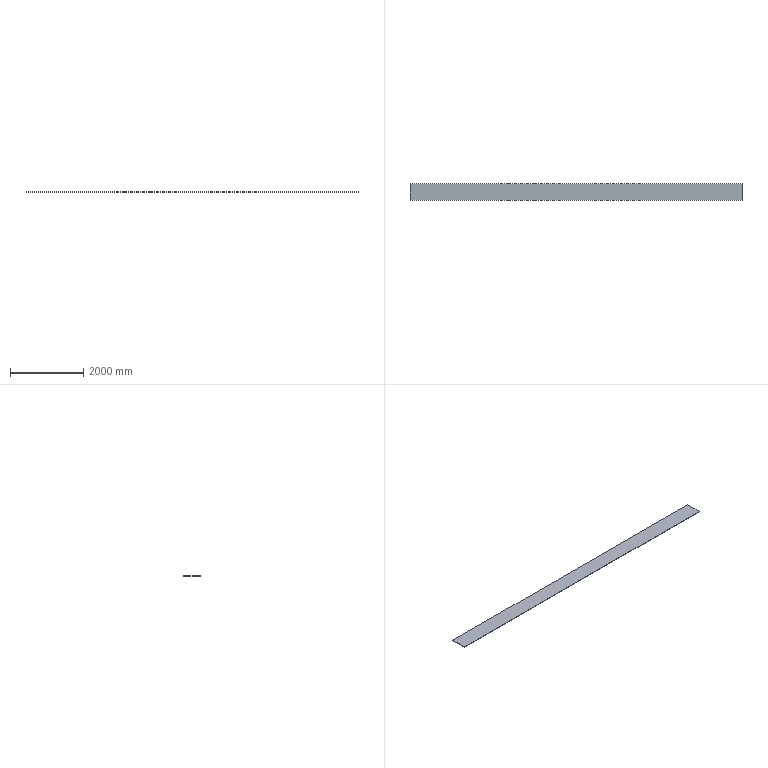Component | SolidWorks | Main-1_9340X450X10-1 | 1 solid | 6 faces | box 9070 x 450 x 10 mm | volume 40815000 mm3 | plane 6 | material Plain Carbon Steel
STEP:
#1=COLOUR_RGB('',0.7922,0.8196,0.9333);
#2=FILL_AREA_STYLE_COLOUR('',#1);
#3=FILL_AREA_STYLE('',(#2));
#4=SURFACE_STYLE_FILL_AREA(#3);
#5=SURFACE_SIDE_STYLE('',(#4));
#6=SURFACE_STYLE_USAGE(.BOTH.,#5);
#7=PRESENTATION_STYLE_ASSIGNMENT((#6));
#8=CARTESIAN_POINT('',(-120.953,84.501,189.605));
#9=VERTEX_POINT('',#8);
#10=CARTESIAN_POINT('',(-120.953,66.784,189.605));
#11=VERTEX_POINT('',#10);
#12=CARTESIAN_POINT('',(-120.953,84.501,189.605));
#13=DIRECTION('',(0.,-1.,-0.));
#14=VECTOR('',#13,39.37);
#15=LINE('',#12,#14);
#16=EDGE_CURVE('',#9,#11,#15,.T.);
#17=ORIENTED_EDGE('',*,*,#16,.F.);
#18=CARTESIAN_POINT('',(-120.953,84.501,189.212));
#19=VERTEX_POINT('',#18);
#20=CARTESIAN_POINT('',(-120.953,84.501,189.212));
#21=DIRECTION('',(0.,-0.,1.));
#22=VECTOR('',#21,39.37);
#23=LINE('',#20,#22);
#24=EDGE_CURVE('',#19,#9,#23,.T.);
#25=ORIENTED_EDGE('',*,*,#24,.F.);
#26=CARTESIAN_POINT('',(-120.953,66.784,189.212));
#27=VERTEX_POINT('',#26);
#28=CARTESIAN_POINT('',(-120.953,84.501,189.212));
#29=DIRECTION('',(0.,-1.,-0.));
#30=VECTOR('',#29,39.37);
#31=LINE('',#28,#30);
#32=EDGE_CURVE('',#19,#27,#31,.T.);
#33=ORIENTED_EDGE('',*,*,#32,.T.);
#34=CARTESIAN_POINT('',(-120.953,66.784,189.212));
#35=DIRECTION('',(0.,-0.,1.));
#36=VECTOR('',#35,39.37);
#37=LINE('',#34,#36);
#38=EDGE_CURVE('',#27,#11,#37,.T.);
#39=ORIENTED_EDGE('',*,*,#38,.T.);
#40=EDGE_LOOP('',(#17,#25,#33,#39));
#41=FACE_OUTER_BOUND('',#40,.T.);
#42=CARTESIAN_POINT('',(-120.953,84.501,189.212));
#43=DIRECTION('',(-1.,-0.,-0.));
#44=DIRECTION('',(0.,-1.,-0.));
#45=AXIS2_PLACEMENT_3D('',#42,#43,#44);
#46=PLANE('',#45);
#47=ADVANCED_FACE('',(#41),#46,.T.);
#48=CARTESIAN_POINT('',(236.134,84.501,189.605));
#49=VERTEX_POINT('',#48);
#50=CARTESIAN_POINT('',(-120.953,84.501,189.605));
#51=DIRECTION('',(-1.,0.,0.));
#52=VECTOR('',#51,39.37);
#53=LINE('',#50,#52);
#54=EDGE_CURVE('',#49,#9,#53,.T.);
#55=ORIENTED_EDGE('',*,*,#54,.F.);
#56=CARTESIAN_POINT('',(236.134,84.501,189.212));
#57=VERTEX_POINT('',#56);
#58=CARTESIAN_POINT('',(236.134,84.501,189.212));
#59=DIRECTION('',(0.,-0.,1.));
#60=VECTOR('',#59,39.37);
#61=LINE('',#58,#60);
#62=EDGE_CURVE('',#57,#49,#61,.T.);
#63=ORIENTED_EDGE('',*,*,#62,.F.);
#64=CARTESIAN_POINT('',(-120.953,84.501,189.212));
#65=DIRECTION('',(-1.,0.,0.));
#66=VECTOR('',#65,39.37);
#67=LINE('',#64,#66);
#68=EDGE_CURVE('',#57,#19,#67,.T.);
#69=ORIENTED_EDGE('',*,*,#68,.T.);
#70=ORIENTED_EDGE('',*,*,#24,.T.);
#71=EDGE_LOOP('',(#55,#63,#69,#70));
#72=FACE_OUTER_BOUND('',#71,.T.);
#73=CARTESIAN_POINT('',(-120.953,84.501,189.212));
#74=DIRECTION('',(0.,1.,0.));
#75=DIRECTION('',(-1.,0.,0.));
#76=AXIS2_PLACEMENT_3D('',#73,#74,#75);
#77=PLANE('',#76);
#78=ADVANCED_FACE('',(#72),#77,.T.);
#79=CARTESIAN_POINT('',(236.134,66.784,189.605));
#80=VERTEX_POINT('',#79);
#81=CARTESIAN_POINT('',(236.134,84.501,189.605));
#82=DIRECTION('',(0.,1.,0.));
#83=VECTOR('',#82,39.37);
#84=LINE('',#81,#83);
#85=EDGE_CURVE('',#80,#49,#84,.T.);
#86=ORIENTED_EDGE('',*,*,#85,.F.);
#87=CARTESIAN_POINT('',(236.134,66.784,189.212));
#88=VERTEX_POINT('',#87);
#89=CARTESIAN_POINT('',(236.134,66.784,189.212));
#90=DIRECTION('',(0.,-0.,1.));
#91=VECTOR('',#90,39.37);
#92=LINE('',#89,#91);
#93=EDGE_CURVE('',#88,#80,#92,.T.);
#94=ORIENTED_EDGE('',*,*,#93,.F.);
#95=CARTESIAN_POINT('',(236.134,84.501,189.212));
#96=DIRECTION('',(0.,1.,0.));
#97=VECTOR('',#96,39.37);
#98=LINE('',#95,#97);
#99=EDGE_CURVE('',#88,#57,#98,.T.);
#100=ORIENTED_EDGE('',*,*,#99,.T.);
#101=ORIENTED_EDGE('',*,*,#62,.T.);
#102=EDGE_LOOP('',(#86,#94,#100,#101));
#103=FACE_OUTER_BOUND('',#102,.T.);
#104=CARTESIAN_POINT('',(236.134,84.501,189.212));
#105=DIRECTION('',(1.,0.,0.));
#106=DIRECTION('',(0.,1.,0.));
#107=AXIS2_PLACEMENT_3D('',#104,#105,#106);
#108=PLANE('',#107);
#109=ADVANCED_FACE('',(#103),#108,.T.);
#110=CARTESIAN_POINT('',(-120.953,66.784,189.605));
#111=DIRECTION('',(1.,0.,0.));
#112=VECTOR('',#111,39.37);
#113=LINE('',#110,#112);
#114=EDGE_CURVE('',#11,#80,#113,.T.);
#115=ORIENTED_EDGE('',*,*,#114,.F.);
#116=ORIENTED_EDGE('',*,*,#38,.F.);
#117=CARTESIAN_POINT('',(-120.953,66.784,189.212));
#118=DIRECTION('',(1.,0.,0.));
#119=VECTOR('',#118,39.37);
#120=LINE('',#117,#119);
#121=EDGE_CURVE('',#27,#88,#120,.T.);
#122=ORIENTED_EDGE('',*,*,#121,.T.);
#123=ORIENTED_EDGE('',*,*,#93,.T.);
#124=EDGE_LOOP('',(#115,#116,#122,#123));
#125=FACE_OUTER_BOUND('',#124,.T.);
#126=CARTESIAN_POINT('',(-120.953,66.784,189.212));
#127=DIRECTION('',(0.,-1.,-0.));
#128=DIRECTION('',(1.,0.,0.));
#129=AXIS2_PLACEMENT_3D('',#126,#127,#128);
#130=PLANE('',#129);
#131=ADVANCED_FACE('',(#125),#130,.T.);
#132=ORIENTED_EDGE('',*,*,#32,.F.);
#133=ORIENTED_EDGE('',*,*,#68,.F.);
#134=ORIENTED_EDGE('',*,*,#99,.F.);
#135=ORIENTED_EDGE('',*,*,#121,.F.);
#136=EDGE_LOOP('',(#132,#133,#134,#135));
#137=FACE_OUTER_BOUND('',#136,.T.);
#138=CARTESIAN_POINT('',(-120.953,84.501,189.212));
#139=DIRECTION('',(0.,-0.,1.));
#140=DIRECTION('',(0.,-1.,-0.));
#141=AXIS2_PLACEMENT_3D('',#138,#139,#140);
#142=PLANE('',#141);
#143=ADVANCED_FACE('',(#137),#142,.F.);
#144=ORIENTED_EDGE('',*,*,#16,.T.);
#145=ORIENTED_EDGE('',*,*,#114,.T.);
#146=ORIENTED_EDGE('',*,*,#85,.T.);
#147=ORIENTED_EDGE('',*,*,#54,.T.);
#148=EDGE_LOOP('',(#144,#145,#146,#147));
#149=FACE_OUTER_BOUND('',#148,.T.);
#150=CARTESIAN_POINT('',(-120.953,84.501,189.605));
#151=DIRECTION('',(0.,-0.,1.));
#152=DIRECTION('',(0.,-1.,-0.));
#153=AXIS2_PLACEMENT_3D('',#150,#151,#152);
#154=PLANE('',#153);
#155=ADVANCED_FACE('',(#149),#154,.T.);
#156=CLOSED_SHELL('',(#47,#78,#109,#131,#143,#155));
#157=MANIFOLD_SOLID_BREP('',#156);
#158=STYLED_ITEM('',(#7),#157);
#159=PRESENTATION_LAYER_ASSIGNMENT('','',(#158));
#160=(LENGTH_UNIT()NAMED_UNIT(*)SI_UNIT($,.METRE.));
#161=LENGTH_MEASURE_WITH_UNIT(LENGTH_MEASURE(0.0254),#160);
#162=DIMENSIONAL_EXPONENTS(1.,0.,0.,0.,0.,0.,0.);
#163=(CONVERSION_BASED_UNIT('',#161)LENGTH_UNIT()NAMED_UNIT(#162));
#164=UNCERTAINTY_MEASURE_WITH_UNIT(LENGTH_MEASURE(0.00001),#163,'','');
#165=(NAMED_UNIT(*)PLANE_ANGLE_UNIT()SI_UNIT($,.RADIAN.));
#166=(NAMED_UNIT(*)SI_UNIT($,.STERADIAN.)SOLID_ANGLE_UNIT());
#167=(GEOMETRIC_REPRESENTATION_CONTEXT(3)GLOBAL_UNCERTAINTY_ASSIGNED_CONTEXT((#164))GLOBAL_UNIT_ASSIGNED_CONTEXT((#163,#165,#166))REPRESENTATION_CONTEXT('',''));
#168=MECHANICAL_DESIGN_GEOMETRIC_PRESENTATION_REPRESENTATION('',(#158),#167);
#169=CARTESIAN_POINT('',(0.,0.,0.));
#170=DIRECTION('',(0.,0.,1.));
#171=DIRECTION('',(1.,0.,0.));
#172=AXIS2_PLACEMENT_3D('',#169,#170,#171);
#173=(LENGTH_UNIT()NAMED_UNIT(*)SI_UNIT($,.METRE.));
#174=LENGTH_MEASURE_WITH_UNIT(LENGTH_MEASURE(0.0254),#173);
#175=DIMENSIONAL_EXPONENTS(1.,0.,0.,0.,0.,0.,0.);
#176=(CONVERSION_BASED_UNIT('',#174)LENGTH_UNIT()NAMED_UNIT(#175));
#177=UNCERTAINTY_MEASURE_WITH_UNIT(LENGTH_MEASURE(0.00001),#176,'','');
#178=(NAMED_UNIT(*)PLANE_ANGLE_UNIT()SI_UNIT($,.RADIAN.));
#179=(NAMED_UNIT(*)SI_UNIT($,.STERADIAN.)SOLID_ANGLE_UNIT());
#180=(GEOMETRIC_REPRESENTATION_CONTEXT(3)GLOBAL_UNCERTAINTY_ASSIGNED_CONTEXT((#177))GLOBAL_UNIT_ASSIGNED_CONTEXT((#176,#178,#179))REPRESENTATION_CONTEXT('',''));
#181=ADVANCED_BREP_SHAPE_REPRESENTATION('',(#157,#172),#180);